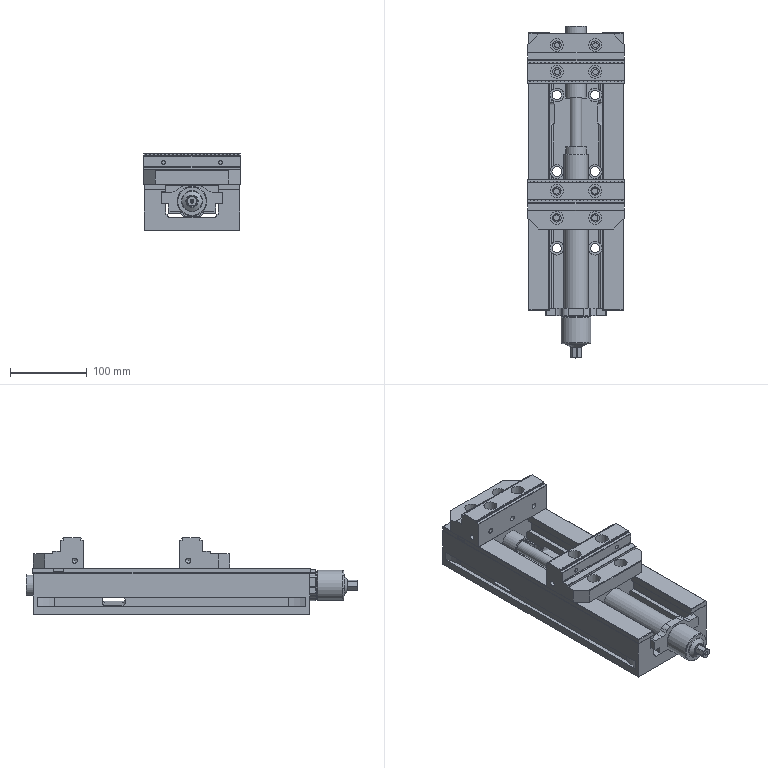Assembly | NX | mm | 7 component files | 7 solids | 884 faces | box 125.4 x 433.44 x 100 mm | volume 2412946 mm3 | plane 593 | cylinder 261 | cone 24 | torus 4 | spline 2 | commonest cylinder face diameters 6 x114 1 x24 12 x16 6.8 x10 18 x9 4 x8 11 x8 17 x8
Bill of materials:
unnamed part 1 | 1 |  | Stepped prismatic block with an L-shaped/stepped end profile, two serrated (scalloped-tooth) edge strips running along its length, four through holes on two stepped top faces, small side holes, and angled chamfers at the corners of one end.
unnamed part 2 | 1 |  | Slender stepped cylindrical, rod-like body of several coaxial diameters: a long main barrel, a thinner rod section extending from one end with a short larger-diameter tip, and a short larger collar plus small pin at the other end.
unnamed part 3 | 1 |  | Rectangular housing block with one large cylindrical bore through its length, a stepped top with a longitudinal rectangular slot/groove dividing it, side ledges/shoulders, chamfered lower corners, and six vertical holes in the top.
unnamed part 4 | 1 |  | Flat plate of even thickness with a central oblong/rounded-rectangle through opening, a widened center region with smooth concave transitions, and narrower rectangular tabs at both ends with chamfered corners.
unnamed part 5 | 1 |  | Long channel/rail body with a U-shaped stepped cross-section: two raised side walls with inner steps/undercuts, a recessed center floor with rounded inner corners, a row of through holes along the floor, small slots on the side face, and notches in the wall tops at one end.
unnamed part 6 | 1 |  | Rectangular block with side shoulders and a top transverse groove, with a cylindrical tube/shaft running through and sticking out from both opposite faces; top face has several small holes and two larger holes.
unnamed part 7 | 1 |  | Stepped prismatic block with an L-shaped/stepped end profile, serrated edge strips along its length, four larger through holes (two partly truncated by a step), three cone-bottomed side holes, and angled corner chamfers on one long edge.
Mates:
1. fix | Clamp_Body_1 1 component
2. center | Clamp_Body_1 1 face | Clamp_Body_1 1 face | Moving_Slider_Other_Half 1 face | Moving_Slider_Other_Half 1 face
3. touch align | Clamp_Body_1 1 face | Moving_Slider_Other_Half 1 face
4. touch align | Moving_Slider_Other_Half 1 face | Clamp_Body_1 1 face
5. center | Moving_Slider 1 face | Moving_Slider 1 face | Clamp_Body_1 1 face | Clamp_Body_1 1 face
6. touch align | Moving_Slider 1 face | Moving_Slider_Other_Half 1 face
7. touch align | gan_1 1 face | Moving_Slider_Other_Half 1 face
8. distance | gan_1 1 face | Moving_Slider_Other_Half 1 face
9. center | Jaw_Fixed_125 1 face | Jaw_Fixed_125 1 face | Clamp_Body_1 1 face | Clamp_Body_1 1 face
10. touch align | Clamp_Body_1 1 face | Jaw_Fixed_125 1 face
11. center | Jaw_Fixed_125 1 face | Jaw_Fixed_125 1 face | Moving_Slider_Other_Half 1 face | Moving_Slider_Other_Half 1 face
12. center | Jaw_Moving_125 1 face | Jaw_Moving_125 1 face | Clamp_Body_1 1 face | Clamp_Body_1 1 face
13. touch align | Clamp_Body_1 1 face | Jaw_Moving_125 1 face
14. touch align | Moving_Slider 1 face | Jaw_Moving_125 1 face
15. center | model20 1 face | model20 1 face | Clamp_Body_1 1 face | Clamp_Body_1 1 face
16. touch align | model20 1 face | Clamp_Body_1 1 face
17. touch align | gan_1 1 face | model20 1 face